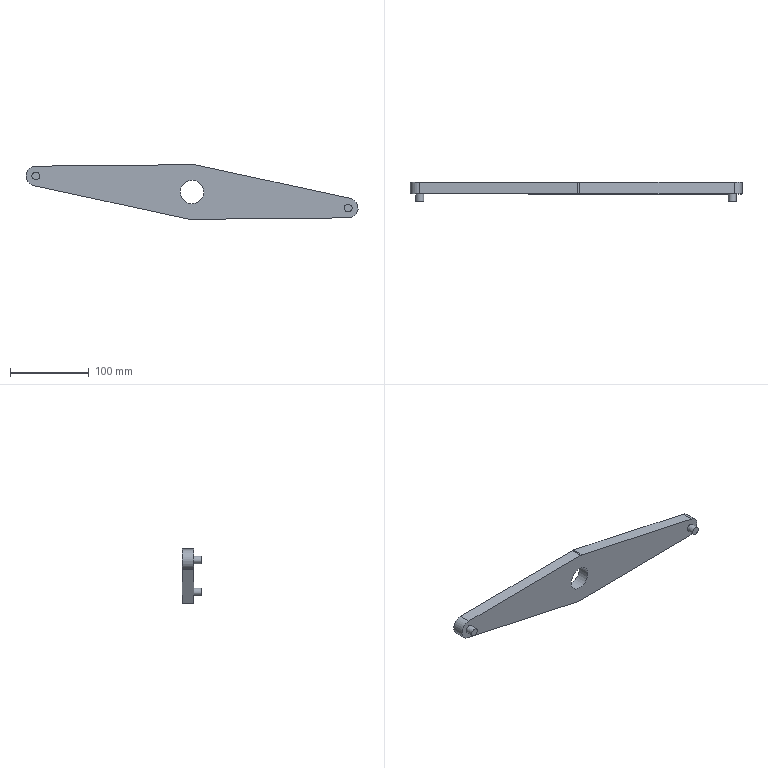Component | NX | 02 | 1 solid | 15 faces | box 422.91 x 25 x 69.61 mm | volume 283802 mm3 | plane 8 | cylinder 7 | commonest cylinder face diameters 25 x2 20 x2 10 x2 30 x1
STEP:
#1=CARTESIAN_POINT('',(0.,0.,0.));
#2=DIRECTION('',(0.,0.,1.));
#3=DIRECTION('',(1.,0.,0.));
#4=AXIS2_PLACEMENT_3D('',#1,#2,#3);
#5=CARTESIAN_POINT('',(-199.074,30.,352.909));
#6=VERTEX_POINT('',#5);
#7=CARTESIAN_POINT('',(-201.609,30.,328.194));
#8=VERTEX_POINT('',#7);
#9=CARTESIAN_POINT('',(-198.956,30.,340.41));
#10=DIRECTION('',(0.,-1.,0.));
#11=DIRECTION('',(-0.9948,0.,0.102));
#12=AXIS2_PLACEMENT_3D('',#9,#10,#11);
#13=CIRCLE('',#12,12.5);
#14=CARTESIAN_POINT('',(-198.956,15.,340.41));
#15=DIRECTION('',(0.,1.,0.));
#16=DIRECTION('',(0.102,0.,0.9948));
#17=AXIS2_PLACEMENT_3D('',#14,#15,#16);
#18=CYLINDRICAL_SURFACE('',#17,12.5);
#19=CARTESIAN_POINT('',(10.996,15.));
#20=DIRECTION('',(-1.,0.));
#21=VECTOR('',#20,1.);
#22=LINE('',#19,#21);
#23=(GEOMETRIC_REPRESENTATION_CONTEXT(2)PARAMETRIC_REPRESENTATION_CONTEXT()REPRESENTATION_CONTEXT('',''));
#24=DEFINITIONAL_REPRESENTATION('',(#22),#23);
#25=PCURVE('',#18,#24);
#26=CARTESIAN_POINT('',(-198.956,30.,340.41));
#27=DIRECTION('',(0.,-1.,0.));
#28=DIRECTION('',(-0.102,0.,-0.9948));
#29=AXIS2_PLACEMENT_3D('',#26,#27,#28);
#30=PLANE('',#29);
#31=CARTESIAN_POINT('',(0.,0.));
#32=DIRECTION('',(-0.,-1.));
#33=AXIS2_PLACEMENT_2D('',#31,#32);
#34=CIRCLE('',#33,12.5);
#35=(GEOMETRIC_REPRESENTATION_CONTEXT(2)PARAMETRIC_REPRESENTATION_CONTEXT()REPRESENTATION_CONTEXT('',''));
#36=DEFINITIONAL_REPRESENTATION('',(#34),#35);
#37=PCURVE('',#30,#36);
#38=SURFACE_CURVE('',#13,(#25,#37),.PCURVE_S1.);
#39=EDGE_CURVE('',#6,#8,#38,.T.);
#40=ORIENTED_EDGE('',*,*,#39,.T.);
#41=CARTESIAN_POINT('',(-201.609,15.,328.194));
#42=VERTEX_POINT('',#41);
#43=CARTESIAN_POINT('',(-201.609,15.,328.194));
#44=DIRECTION('',(0.,1.,0.));
#45=VECTOR('',#44,1.);
#46=LINE('',#43,#45);
#47=CARTESIAN_POINT('',(3.253,0.));
#48=DIRECTION('',(0.,1.));
#49=VECTOR('',#48,1.);
#50=LINE('',#47,#49);
#51=(GEOMETRIC_REPRESENTATION_CONTEXT(2)PARAMETRIC_REPRESENTATION_CONTEXT()REPRESENTATION_CONTEXT('',''));
#52=DEFINITIONAL_REPRESENTATION('',(#50),#51);
#53=PCURVE('',#18,#52);
#54=CARTESIAN_POINT('',(-201.609,15.,328.194));
#55=DIRECTION('',(0.2122,0.,0.9772));
#56=DIRECTION('',(0.9772,0.,-0.2122));
#57=AXIS2_PLACEMENT_3D('',#54,#55,#56);
#58=PLANE('',#57);
#59=CARTESIAN_POINT('',(0.,0.));
#60=DIRECTION('',(0.,1.));
#61=VECTOR('',#60,1.);
#62=LINE('',#59,#61);
#63=(GEOMETRIC_REPRESENTATION_CONTEXT(2)PARAMETRIC_REPRESENTATION_CONTEXT()REPRESENTATION_CONTEXT('',''));
#64=DEFINITIONAL_REPRESENTATION('',(#62),#63);
#65=PCURVE('',#58,#64);
#66=SURFACE_CURVE('',#46,(#53,#65),.PCURVE_S1.);
#67=EDGE_CURVE('',#42,#8,#66,.T.);
#68=ORIENTED_EDGE('',*,*,#67,.F.);
#69=CARTESIAN_POINT('',(-199.074,15.,352.909));
#70=VERTEX_POINT('',#69);
#71=CARTESIAN_POINT('',(-198.956,15.,340.41));
#72=DIRECTION('',(0.,-1.,0.));
#73=DIRECTION('',(-0.9948,0.,0.102));
#74=AXIS2_PLACEMENT_3D('',#71,#72,#73);
#75=CIRCLE('',#74,12.5);
#76=CARTESIAN_POINT('',(10.996,0.));
#77=DIRECTION('',(-1.,0.));
#78=VECTOR('',#77,1.);
#79=LINE('',#76,#78);
#80=(GEOMETRIC_REPRESENTATION_CONTEXT(2)PARAMETRIC_REPRESENTATION_CONTEXT()REPRESENTATION_CONTEXT('',''));
#81=DEFINITIONAL_REPRESENTATION('',(#79),#80);
#82=PCURVE('',#18,#81);
#83=CARTESIAN_POINT('',(-198.956,15.,340.41));
#84=DIRECTION('',(0.,-1.,0.));
#85=DIRECTION('',(-0.102,0.,-0.9948));
#86=AXIS2_PLACEMENT_3D('',#83,#84,#85);
#87=PLANE('',#86);
#88=CARTESIAN_POINT('',(0.,0.));
#89=DIRECTION('',(-0.,-1.));
#90=AXIS2_PLACEMENT_2D('',#88,#89);
#91=CIRCLE('',#90,12.5);
#92=(GEOMETRIC_REPRESENTATION_CONTEXT(2)PARAMETRIC_REPRESENTATION_CONTEXT()REPRESENTATION_CONTEXT('',''));
#93=DEFINITIONAL_REPRESENTATION('',(#91),#92);
#94=PCURVE('',#87,#93);
#95=SURFACE_CURVE('',#75,(#82,#94),.PCURVE_S1.);
#96=EDGE_CURVE('',#70,#42,#95,.T.);
#97=ORIENTED_EDGE('',*,*,#96,.F.);
#98=CARTESIAN_POINT('',(-199.074,15.,352.909));
#99=DIRECTION('',(0.,1.,0.));
#100=VECTOR('',#99,1.);
#101=LINE('',#98,#100);
#102=CARTESIAN_POINT('',(6.172,0.));
#103=DIRECTION('',(0.,1.));
#104=VECTOR('',#103,1.);
#105=LINE('',#102,#104);
#106=(GEOMETRIC_REPRESENTATION_CONTEXT(2)PARAMETRIC_REPRESENTATION_CONTEXT()REPRESENTATION_CONTEXT('',''));
#107=DEFINITIONAL_REPRESENTATION('',(#105),#106);
#108=PCURVE('',#18,#107);
#109=CARTESIAN_POINT('',(3.572,15.,354.817));
#110=DIRECTION('',(0.009416,0.,-1.));
#111=DIRECTION('',(-1.,0.,-0.009416));
#112=AXIS2_PLACEMENT_3D('',#109,#110,#111);
#113=PLANE('',#112);
#114=CARTESIAN_POINT('',(202.654,0.));
#115=DIRECTION('',(0.,1.));
#116=VECTOR('',#115,1.);
#117=LINE('',#114,#116);
#118=(GEOMETRIC_REPRESENTATION_CONTEXT(2)PARAMETRIC_REPRESENTATION_CONTEXT()REPRESENTATION_CONTEXT('',''));
#119=DEFINITIONAL_REPRESENTATION('',(#117),#118);
#120=PCURVE('',#113,#119);
#121=SURFACE_CURVE('',#101,(#108,#120),.PCURVE_S1.);
#122=EDGE_CURVE('',#70,#6,#121,.T.);
#123=ORIENTED_EDGE('',*,*,#122,.T.);
#124=EDGE_LOOP('',(#40,#68,#97,#123));
#125=FACE_BOUND('',#124,.T.);
#126=ADVANCED_FACE('',(#125),#18,.T.);
#127=CARTESIAN_POINT('',(-4.667,30.,285.421));
#128=VERTEX_POINT('',#127);
#129=CARTESIAN_POINT('',(-201.609,30.,328.194));
#130=DIRECTION('',(0.9772,0.,-0.2122));
#131=VECTOR('',#130,1.);
#132=LINE('',#129,#131);
#133=CARTESIAN_POINT('',(0.,15.));
#134=DIRECTION('',(1.,0.));
#135=VECTOR('',#134,1.);
#136=LINE('',#133,#135);
#137=(GEOMETRIC_REPRESENTATION_CONTEXT(2)PARAMETRIC_REPRESENTATION_CONTEXT()REPRESENTATION_CONTEXT('',''));
#138=DEFINITIONAL_REPRESENTATION('',(#136),#137);
#139=PCURVE('',#58,#138);
#140=CARTESIAN_POINT('',(12.422,-1.393));
#141=DIRECTION('',(0.1114,0.9938));
#142=VECTOR('',#141,1.);
#143=LINE('',#140,#142);
#144=(GEOMETRIC_REPRESENTATION_CONTEXT(2)PARAMETRIC_REPRESENTATION_CONTEXT()REPRESENTATION_CONTEXT('',''));
#145=DEFINITIONAL_REPRESENTATION('',(#143),#144);
#146=PCURVE('',#30,#145);
#147=SURFACE_CURVE('',#132,(#139,#146),.PCURVE_S1.);
#148=EDGE_CURVE('',#8,#128,#147,.T.);
#149=ORIENTED_EDGE('',*,*,#148,.T.);
#150=CARTESIAN_POINT('',(-4.667,15.,285.421));
#151=VERTEX_POINT('',#150);
#152=CARTESIAN_POINT('',(-4.667,15.,285.421));
#153=DIRECTION('',(0.,-1.,0.));
#154=VECTOR('',#153,1.);
#155=LINE('',#152,#154);
#156=CARTESIAN_POINT('',(201.533,0.));
#157=DIRECTION('',(0.,-1.));
#158=VECTOR('',#157,1.);
#159=LINE('',#156,#158);
#160=(GEOMETRIC_REPRESENTATION_CONTEXT(2)PARAMETRIC_REPRESENTATION_CONTEXT()REPRESENTATION_CONTEXT('',''));
#161=DEFINITIONAL_REPRESENTATION('',(#159),#160);
#162=PCURVE('',#58,#161);
#163=CARTESIAN_POINT('',(-2.545,15.,295.193));
#164=DIRECTION('',(0.,1.,0.));
#165=DIRECTION('',(0.102,0.,0.9948));
#166=AXIS2_PLACEMENT_3D('',#163,#164,#165);
#167=CYLINDRICAL_SURFACE('',#166,10.);
#168=CARTESIAN_POINT('',(3.253,0.));
#169=DIRECTION('',(0.,-1.));
#170=VECTOR('',#169,1.);
#171=LINE('',#168,#170);
#172=(GEOMETRIC_REPRESENTATION_CONTEXT(2)PARAMETRIC_REPRESENTATION_CONTEXT()REPRESENTATION_CONTEXT('',''));
#173=DEFINITIONAL_REPRESENTATION('',(#171),#172);
#174=PCURVE('',#167,#173);
#175=SURFACE_CURVE('',#155,(#162,#174),.PCURVE_S1.);
#176=EDGE_CURVE('',#128,#151,#175,.T.);
#177=ORIENTED_EDGE('',*,*,#176,.T.);
#178=CARTESIAN_POINT('',(-201.609,15.,328.194));
#179=DIRECTION('',(0.9772,0.,-0.2122));
#180=VECTOR('',#179,1.);
#181=LINE('',#178,#180);
#182=CARTESIAN_POINT('',(0.,0.));
#183=DIRECTION('',(1.,0.));
#184=VECTOR('',#183,1.);
#185=LINE('',#182,#184);
#186=(GEOMETRIC_REPRESENTATION_CONTEXT(2)PARAMETRIC_REPRESENTATION_CONTEXT()REPRESENTATION_CONTEXT('',''));
#187=DEFINITIONAL_REPRESENTATION('',(#185),#186);
#188=PCURVE('',#58,#187);
#189=CARTESIAN_POINT('',(12.422,-1.393));
#190=DIRECTION('',(0.1114,0.9938));
#191=VECTOR('',#190,1.);
#192=LINE('',#189,#191);
#193=(GEOMETRIC_REPRESENTATION_CONTEXT(2)PARAMETRIC_REPRESENTATION_CONTEXT()REPRESENTATION_CONTEXT('',''));
#194=DEFINITIONAL_REPRESENTATION('',(#192),#193);
#195=PCURVE('',#87,#194);
#196=SURFACE_CURVE('',#181,(#188,#195),.PCURVE_S1.);
#197=EDGE_CURVE('',#42,#151,#196,.T.);
#198=ORIENTED_EDGE('',*,*,#197,.F.);
#199=ORIENTED_EDGE('',*,*,#67,.T.);
#200=EDGE_LOOP('',(#149,#177,#198,#199));
#201=FACE_BOUND('',#200,.T.);
#202=ADVANCED_FACE('',(#201),#58,.F.);
#203=CARTESIAN_POINT('',(-2.451,15.,285.193));
#204=VERTEX_POINT('',#203);
#205=CARTESIAN_POINT('',(199.074,15.,287.091));
#206=VERTEX_POINT('',#205);
#207=CARTESIAN_POINT('',(-3.572,15.,285.183));
#208=DIRECTION('',(1.,0.,0.009416));
#209=VECTOR('',#208,1.);
#210=LINE('',#207,#209);
#211=CARTESIAN_POINT('',(-3.572,15.,285.183));
#212=DIRECTION('',(-0.009416,0.,1.));
#213=DIRECTION('',(1.,0.,0.009416));
#214=AXIS2_PLACEMENT_3D('',#211,#212,#213);
#215=PLANE('',#214);
#216=CARTESIAN_POINT('',(0.,0.));
#217=DIRECTION('',(1.,0.));
#218=VECTOR('',#217,1.);
#219=LINE('',#216,#218);
#220=(GEOMETRIC_REPRESENTATION_CONTEXT(2)PARAMETRIC_REPRESENTATION_CONTEXT()REPRESENTATION_CONTEXT('',''));
#221=DEFINITIONAL_REPRESENTATION('',(#219),#220);
#222=PCURVE('',#215,#221);
#223=CARTESIAN_POINT('',(35.,200.));
#224=DIRECTION('',(-0.1114,0.9938));
#225=VECTOR('',#224,1.);
#226=LINE('',#223,#225);
#227=(GEOMETRIC_REPRESENTATION_CONTEXT(2)PARAMETRIC_REPRESENTATION_CONTEXT()REPRESENTATION_CONTEXT('',''));
#228=DEFINITIONAL_REPRESENTATION('',(#226),#227);
#229=PCURVE('',#87,#228);
#230=SURFACE_CURVE('',#210,(#222,#229),.PCURVE_S1.);
#231=EDGE_CURVE('',#204,#206,#230,.T.);
#232=ORIENTED_EDGE('',*,*,#231,.F.);
#233=CARTESIAN_POINT('',(-2.451,30.,285.193));
#234=VERTEX_POINT('',#233);
#235=CARTESIAN_POINT('',(-2.451,15.,285.193));
#236=DIRECTION('',(0.,1.,0.));
#237=VECTOR('',#236,1.);
#238=LINE('',#235,#237);
#239=CARTESIAN_POINT('',(1.121,0.));
#240=DIRECTION('',(0.,1.));
#241=VECTOR('',#240,1.);
#242=LINE('',#239,#241);
#243=(GEOMETRIC_REPRESENTATION_CONTEXT(2)PARAMETRIC_REPRESENTATION_CONTEXT()REPRESENTATION_CONTEXT('',''));
#244=DEFINITIONAL_REPRESENTATION('',(#242),#243);
#245=PCURVE('',#215,#244);
#246=CARTESIAN_POINT('',(3.03,0.));
#247=DIRECTION('',(0.,1.));
#248=VECTOR('',#247,1.);
#249=LINE('',#246,#248);
#250=(GEOMETRIC_REPRESENTATION_CONTEXT(2)PARAMETRIC_REPRESENTATION_CONTEXT()REPRESENTATION_CONTEXT('',''));
#251=DEFINITIONAL_REPRESENTATION('',(#249),#250);
#252=PCURVE('',#167,#251);
#253=SURFACE_CURVE('',#238,(#245,#252),.PCURVE_S1.);
#254=EDGE_CURVE('',#204,#234,#253,.T.);
#255=ORIENTED_EDGE('',*,*,#254,.T.);
#256=CARTESIAN_POINT('',(199.074,30.,287.091));
#257=VERTEX_POINT('',#256);
#258=CARTESIAN_POINT('',(-3.572,30.,285.183));
#259=DIRECTION('',(1.,0.,0.009416));
#260=VECTOR('',#259,1.);
#261=LINE('',#258,#260);
#262=CARTESIAN_POINT('',(0.,15.));
#263=DIRECTION('',(1.,0.));
#264=VECTOR('',#263,1.);
#265=LINE('',#262,#264);
#266=(GEOMETRIC_REPRESENTATION_CONTEXT(2)PARAMETRIC_REPRESENTATION_CONTEXT()REPRESENTATION_CONTEXT('',''));
#267=DEFINITIONAL_REPRESENTATION('',(#265),#266);
#268=PCURVE('',#215,#267);
#269=CARTESIAN_POINT('',(35.,200.));
#270=DIRECTION('',(-0.1114,0.9938));
#271=VECTOR('',#270,1.);
#272=LINE('',#269,#271);
#273=(GEOMETRIC_REPRESENTATION_CONTEXT(2)PARAMETRIC_REPRESENTATION_CONTEXT()REPRESENTATION_CONTEXT('',''));
#274=DEFINITIONAL_REPRESENTATION('',(#272),#273);
#275=PCURVE('',#30,#274);
#276=SURFACE_CURVE('',#261,(#268,#275),.PCURVE_S1.);
#277=EDGE_CURVE('',#234,#257,#276,.T.);
#278=ORIENTED_EDGE('',*,*,#277,.T.);
#279=CARTESIAN_POINT('',(199.074,15.,287.091));
#280=DIRECTION('',(0.,1.,0.));
#281=VECTOR('',#280,1.);
#282=LINE('',#279,#281);
#283=CARTESIAN_POINT('',(202.654,0.));
#284=DIRECTION('',(0.,1.));
#285=VECTOR('',#284,1.);
#286=LINE('',#283,#285);
#287=(GEOMETRIC_REPRESENTATION_CONTEXT(2)PARAMETRIC_REPRESENTATION_CONTEXT()REPRESENTATION_CONTEXT('',''));
#288=DEFINITIONAL_REPRESENTATION('',(#286),#287);
#289=PCURVE('',#215,#288);
#290=CARTESIAN_POINT('',(198.956,15.,299.59));
#291=DIRECTION('',(0.,1.,0.));
#292=DIRECTION('',(0.102,0.,0.9948));
#293=AXIS2_PLACEMENT_3D('',#290,#291,#292);
#294=CYLINDRICAL_SURFACE('',#293,12.5);
#295=CARTESIAN_POINT('',(3.03,0.));
#296=DIRECTION('',(0.,1.));
#297=VECTOR('',#296,1.);
#298=LINE('',#295,#297);
#299=(GEOMETRIC_REPRESENTATION_CONTEXT(2)PARAMETRIC_REPRESENTATION_CONTEXT()REPRESENTATION_CONTEXT('',''));
#300=DEFINITIONAL_REPRESENTATION('',(#298),#299);
#301=PCURVE('',#294,#300);
#302=SURFACE_CURVE('',#282,(#289,#301),.PCURVE_S1.);
#303=EDGE_CURVE('',#206,#257,#302,.T.);
#304=ORIENTED_EDGE('',*,*,#303,.F.);
#305=EDGE_LOOP('',(#232,#255,#278,#304));
#306=FACE_BOUND('',#305,.T.);
#307=ADVANCED_FACE('',(#306),#215,.F.);
#308=CARTESIAN_POINT('',(201.609,30.,311.806));
#309=VERTEX_POINT('',#308);
#310=CARTESIAN_POINT('',(198.956,30.,299.59));
#311=DIRECTION('',(0.,-1.,0.));
#312=DIRECTION('',(0.9948,0.,-0.102));
#313=AXIS2_PLACEMENT_3D('',#310,#311,#312);
#314=CIRCLE('',#313,12.5);
#315=CARTESIAN_POINT('',(7.854,15.));
#316=DIRECTION('',(-1.,0.));
#317=VECTOR('',#316,1.);
#318=LINE('',#315,#317);
#319=(GEOMETRIC_REPRESENTATION_CONTEXT(2)PARAMETRIC_REPRESENTATION_CONTEXT()REPRESENTATION_CONTEXT('',''));
#320=DEFINITIONAL_REPRESENTATION('',(#318),#319);
#321=PCURVE('',#294,#320);
#322=CARTESIAN_POINT('',(-0.,400.));
#323=DIRECTION('',(0.,1.));
#324=AXIS2_PLACEMENT_2D('',#322,#323);
#325=CIRCLE('',#324,12.5);
#326=(GEOMETRIC_REPRESENTATION_CONTEXT(2)PARAMETRIC_REPRESENTATION_CONTEXT()REPRESENTATION_CONTEXT('',''));
#327=DEFINITIONAL_REPRESENTATION('',(#325),#326);
#328=PCURVE('',#30,#327);
#329=SURFACE_CURVE('',#314,(#321,#328),.PCURVE_S1.);
#330=EDGE_CURVE('',#257,#309,#329,.T.);
#331=ORIENTED_EDGE('',*,*,#330,.T.);
#332=CARTESIAN_POINT('',(201.609,15.,311.806));
#333=VERTEX_POINT('',#332);
#334=CARTESIAN_POINT('',(201.609,15.,311.806));
#335=DIRECTION('',(0.,1.,0.));
#336=VECTOR('',#335,1.);
#337=LINE('',#334,#336);
#338=CARTESIAN_POINT('',(0.1116,0.));
#339=DIRECTION('',(0.,1.));
#340=VECTOR('',#339,1.);
#341=LINE('',#338,#340);
#342=(GEOMETRIC_REPRESENTATION_CONTEXT(2)PARAMETRIC_REPRESENTATION_CONTEXT()REPRESENTATION_CONTEXT('',''));
#343=DEFINITIONAL_REPRESENTATION('',(#341),#342);
#344=PCURVE('',#294,#343);
#345=CARTESIAN_POINT('',(201.609,15.,311.806));
#346=DIRECTION('',(-0.2122,0.,-0.9772));
#347=DIRECTION('',(-0.9772,0.,0.2122));
#348=AXIS2_PLACEMENT_3D('',#345,#346,#347);
#349=PLANE('',#348);
#350=CARTESIAN_POINT('',(0.,0.));
#351=DIRECTION('',(0.,1.));
#352=VECTOR('',#351,1.);
#353=LINE('',#350,#352);
#354=(GEOMETRIC_REPRESENTATION_CONTEXT(2)PARAMETRIC_REPRESENTATION_CONTEXT()REPRESENTATION_CONTEXT('',''));
#355=DEFINITIONAL_REPRESENTATION('',(#353),#354);
#356=PCURVE('',#349,#355);
#357=SURFACE_CURVE('',#337,(#344,#356),.PCURVE_S1.);
#358=EDGE_CURVE('',#333,#309,#357,.T.);
#359=ORIENTED_EDGE('',*,*,#358,.F.);
#360=CARTESIAN_POINT('',(198.956,15.,299.59));
#361=DIRECTION('',(0.,-1.,0.));
#362=DIRECTION('',(0.9948,0.,-0.102));
#363=AXIS2_PLACEMENT_3D('',#360,#361,#362);
#364=CIRCLE('',#363,12.5);
#365=CARTESIAN_POINT('',(7.854,0.));
#366=DIRECTION('',(-1.,0.));
#367=VECTOR('',#366,1.);
#368=LINE('',#365,#367);
#369=(GEOMETRIC_REPRESENTATION_CONTEXT(2)PARAMETRIC_REPRESENTATION_CONTEXT()REPRESENTATION_CONTEXT('',''));
#370=DEFINITIONAL_REPRESENTATION('',(#368),#369);
#371=PCURVE('',#294,#370);
#372=CARTESIAN_POINT('',(-0.,400.));
#373=DIRECTION('',(0.,1.));
#374=AXIS2_PLACEMENT_2D('',#372,#373);
#375=CIRCLE('',#374,12.5);
#376=(GEOMETRIC_REPRESENTATION_CONTEXT(2)PARAMETRIC_REPRESENTATION_CONTEXT()REPRESENTATION_CONTEXT('',''));
#377=DEFINITIONAL_REPRESENTATION('',(#375),#376);
#378=PCURVE('',#87,#377);
#379=SURFACE_CURVE('',#364,(#371,#378),.PCURVE_S1.);
#380=EDGE_CURVE('',#206,#333,#379,.T.);
#381=ORIENTED_EDGE('',*,*,#380,.F.);
#382=ORIENTED_EDGE('',*,*,#303,.T.);
#383=EDGE_LOOP('',(#331,#359,#381,#382));
#384=FACE_BOUND('',#383,.T.);
#385=ADVANCED_FACE('',(#384),#294,.T.);
#386=CARTESIAN_POINT('',(4.667,30.,354.579));
#387=VERTEX_POINT('',#386);
#388=CARTESIAN_POINT('',(201.609,30.,311.806));
#389=DIRECTION('',(-0.9772,0.,0.2122));
#390=VECTOR('',#389,1.);
#391=LINE('',#388,#390);
#392=CARTESIAN_POINT('',(0.,15.));
#393=DIRECTION('',(1.,0.));
#394=VECTOR('',#393,1.);
#395=LINE('',#392,#394);
#396=(GEOMETRIC_REPRESENTATION_CONTEXT(2)PARAMETRIC_REPRESENTATION_CONTEXT()REPRESENTATION_CONTEXT('',''));
#397=DEFINITIONAL_REPRESENTATION('',(#395),#396);
#398=PCURVE('',#349,#397);
#399=CARTESIAN_POINT('',(-12.422,401.393));
#400=DIRECTION('',(-0.1114,-0.9938));
#401=VECTOR('',#400,1.);
#402=LINE('',#399,#401);
#403=(GEOMETRIC_REPRESENTATION_CONTEXT(2)PARAMETRIC_REPRESENTATION_CONTEXT()REPRESENTATION_CONTEXT('',''));
#404=DEFINITIONAL_REPRESENTATION('',(#402),#403);
#405=PCURVE('',#30,#404);
#406=SURFACE_CURVE('',#391,(#398,#405),.PCURVE_S1.);
#407=EDGE_CURVE('',#309,#387,#406,.T.);
#408=ORIENTED_EDGE('',*,*,#407,.T.);
#409=CARTESIAN_POINT('',(4.667,15.,354.579));
#410=VERTEX_POINT('',#409);
#411=CARTESIAN_POINT('',(4.667,15.,354.579));
#412=DIRECTION('',(0.,-1.,0.));
#413=VECTOR('',#412,1.);
#414=LINE('',#411,#413);
#415=CARTESIAN_POINT('',(201.533,0.));
#416=DIRECTION('',(0.,-1.));
#417=VECTOR('',#416,1.);
#418=LINE('',#415,#417);
#419=(GEOMETRIC_REPRESENTATION_CONTEXT(2)PARAMETRIC_REPRESENTATION_CONTEXT()REPRESENTATION_CONTEXT('',''));
#420=DEFINITIONAL_REPRESENTATION('',(#418),#419);
#421=PCURVE('',#349,#420);
#422=CARTESIAN_POINT('',(2.545,15.,344.807));
#423=DIRECTION('',(0.,1.,0.));
#424=DIRECTION('',(0.102,0.,0.9948));
#425=AXIS2_PLACEMENT_3D('',#422,#423,#424);
#426=CYLINDRICAL_SURFACE('',#425,10.);
#427=CARTESIAN_POINT('',(0.1116,0.));
#428=DIRECTION('',(0.,-1.));
#429=VECTOR('',#428,1.);
#430=LINE('',#427,#429);
#431=(GEOMETRIC_REPRESENTATION_CONTEXT(2)PARAMETRIC_REPRESENTATION_CONTEXT()REPRESENTATION_CONTEXT('',''));
#432=DEFINITIONAL_REPRESENTATION('',(#430),#431);
#433=PCURVE('',#426,#432);
#434=SURFACE_CURVE('',#414,(#421,#433),.PCURVE_S1.);
#435=EDGE_CURVE('',#387,#410,#434,.T.);
#436=ORIENTED_EDGE('',*,*,#435,.T.);
#437=CARTESIAN_POINT('',(201.609,15.,311.806));
#438=DIRECTION('',(-0.9772,0.,0.2122));
#439=VECTOR('',#438,1.);
#440=LINE('',#437,#439);
#441=CARTESIAN_POINT('',(0.,0.));
#442=DIRECTION('',(1.,0.));
#443=VECTOR('',#442,1.);
#444=LINE('',#441,#443);
#445=(GEOMETRIC_REPRESENTATION_CONTEXT(2)PARAMETRIC_REPRESENTATION_CONTEXT()REPRESENTATION_CONTEXT('',''));
#446=DEFINITIONAL_REPRESENTATION('',(#444),#445);
#447=PCURVE('',#349,#446);
#448=CARTESIAN_POINT('',(-12.422,401.393));
#449=DIRECTION('',(-0.1114,-0.9938));
#450=VECTOR('',#449,1.);
#451=LINE('',#448,#450);
#452=(GEOMETRIC_REPRESENTATION_CONTEXT(2)PARAMETRIC_REPRESENTATION_CONTEXT()REPRESENTATION_CONTEXT('',''));
#453=DEFINITIONAL_REPRESENTATION('',(#451),#452);
#454=PCURVE('',#87,#453);
#455=SURFACE_CURVE('',#440,(#447,#454),.PCURVE_S1.);
#456=EDGE_CURVE('',#333,#410,#455,.T.);
#457=ORIENTED_EDGE('',*,*,#456,.F.);
#458=ORIENTED_EDGE('',*,*,#358,.T.);
#459=EDGE_LOOP('',(#408,#436,#457,#458));
#460=FACE_BOUND('',#459,.T.);
#461=ADVANCED_FACE('',(#460),#349,.F.);
#462=CARTESIAN_POINT('',(2.451,15.,354.807));
#463=VERTEX_POINT('',#462);
#464=CARTESIAN_POINT('',(3.572,15.,354.817));
#465=DIRECTION('',(-1.,0.,-0.009416));
#466=VECTOR('',#465,1.);
#467=LINE('',#464,#466);
#468=CARTESIAN_POINT('',(0.,0.));
#469=DIRECTION('',(1.,0.));
#470=VECTOR('',#469,1.);
#471=LINE('',#468,#470);
#472=(GEOMETRIC_REPRESENTATION_CONTEXT(2)PARAMETRIC_REPRESENTATION_CONTEXT()REPRESENTATION_CONTEXT('',''));
#473=DEFINITIONAL_REPRESENTATION('',(#471),#472);
#474=PCURVE('',#113,#473);
#475=CARTESIAN_POINT('',(-35.,200.));
#476=DIRECTION('',(0.1114,-0.9938));
#477=VECTOR('',#476,1.);
#478=LINE('',#475,#477);
#479=(GEOMETRIC_REPRESENTATION_CONTEXT(2)PARAMETRIC_REPRESENTATION_CONTEXT()REPRESENTATION_CONTEXT('',''));
#480=DEFINITIONAL_REPRESENTATION('',(#478),#479);
#481=PCURVE('',#87,#480);
#482=SURFACE_CURVE('',#467,(#474,#481),.PCURVE_S1.);
#483=EDGE_CURVE('',#463,#70,#482,.T.);
#484=ORIENTED_EDGE('',*,*,#483,.F.);
#485=CARTESIAN_POINT('',(2.451,30.,354.807));
#486=VERTEX_POINT('',#485);
#487=CARTESIAN_POINT('',(2.451,15.,354.807));
#488=DIRECTION('',(0.,1.,0.));
#489=VECTOR('',#488,1.);
#490=LINE('',#487,#489);
#491=CARTESIAN_POINT('',(1.121,0.));
#492=DIRECTION('',(0.,1.));
#493=VECTOR('',#492,1.);
#494=LINE('',#491,#493);
#495=(GEOMETRIC_REPRESENTATION_CONTEXT(2)PARAMETRIC_REPRESENTATION_CONTEXT()REPRESENTATION_CONTEXT('',''));
#496=DEFINITIONAL_REPRESENTATION('',(#494),#495);
#497=PCURVE('',#113,#496);
#498=CARTESIAN_POINT('',(-0.1116,0.));
#499=DIRECTION('',(0.,1.));
#500=VECTOR('',#499,1.);
#501=LINE('',#498,#500);
#502=(GEOMETRIC_REPRESENTATION_CONTEXT(2)PARAMETRIC_REPRESENTATION_CONTEXT()REPRESENTATION_CONTEXT('',''));
#503=DEFINITIONAL_REPRESENTATION('',(#501),#502);
#504=PCURVE('',#426,#503);
#505=SURFACE_CURVE('',#490,(#497,#504),.PCURVE_S1.);
#506=EDGE_CURVE('',#463,#486,#505,.T.);
#507=ORIENTED_EDGE('',*,*,#506,.T.);
#508=CARTESIAN_POINT('',(3.572,30.,354.817));
#509=DIRECTION('',(-1.,0.,-0.009416));
#510=VECTOR('',#509,1.);
#511=LINE('',#508,#510);
#512=CARTESIAN_POINT('',(0.,15.));
#513=DIRECTION('',(1.,0.));
#514=VECTOR('',#513,1.);
#515=LINE('',#512,#514);
#516=(GEOMETRIC_REPRESENTATION_CONTEXT(2)PARAMETRIC_REPRESENTATION_CONTEXT()REPRESENTATION_CONTEXT('',''));
#517=DEFINITIONAL_REPRESENTATION('',(#515),#516);
#518=PCURVE('',#113,#517);
#519=CARTESIAN_POINT('',(-35.,200.));
#520=DIRECTION('',(0.1114,-0.9938));
#521=VECTOR('',#520,1.);
#522=LINE('',#519,#521);
#523=(GEOMETRIC_REPRESENTATION_CONTEXT(2)PARAMETRIC_REPRESENTATION_CONTEXT()REPRESENTATION_CONTEXT('',''));
#524=DEFINITIONAL_REPRESENTATION('',(#522),#523);
#525=PCURVE('',#30,#524);
#526=SURFACE_CURVE('',#511,(#518,#525),.PCURVE_S1.);
#527=EDGE_CURVE('',#486,#6,#526,.T.);
#528=ORIENTED_EDGE('',*,*,#527,.T.);
#529=ORIENTED_EDGE('',*,*,#122,.F.);
#530=EDGE_LOOP('',(#484,#507,#528,#529));
#531=FACE_BOUND('',#530,.T.);
#532=ADVANCED_FACE('',(#531),#113,.F.);
#533=CARTESIAN_POINT('',(203.93,15.,299.08));
#534=VERTEX_POINT('',#533);
#535=CARTESIAN_POINT('',(198.956,15.,299.59));
#536=DIRECTION('',(0.,-1.,0.));
#537=DIRECTION('',(0.9948,0.,-0.102));
#538=AXIS2_PLACEMENT_3D('',#535,#536,#537);
#539=CIRCLE('',#538,5.);
#540=CARTESIAN_POINT('',(-0.,400.));
#541=DIRECTION('',(-0.,1.));
#542=AXIS2_PLACEMENT_2D('',#540,#541);
#543=CIRCLE('',#542,5.);
#544=(GEOMETRIC_REPRESENTATION_CONTEXT(2)PARAMETRIC_REPRESENTATION_CONTEXT()REPRESENTATION_CONTEXT('',''));
#545=DEFINITIONAL_REPRESENTATION('',(#543),#544);
#546=PCURVE('',#87,#545);
#547=CARTESIAN_POINT('',(198.956,5.,299.59));
#548=DIRECTION('',(0.,1.,0.));
#549=DIRECTION('',(0.102,0.,0.9948));
#550=AXIS2_PLACEMENT_3D('',#547,#548,#549);
#551=CYLINDRICAL_SURFACE('',#550,5.);
#552=CARTESIAN_POINT('',(7.854,10.));
#553=DIRECTION('',(-1.,0.));
#554=VECTOR('',#553,1.);
#555=LINE('',#552,#554);
#556=(GEOMETRIC_REPRESENTATION_CONTEXT(2)PARAMETRIC_REPRESENTATION_CONTEXT()REPRESENTATION_CONTEXT('',''));
#557=DEFINITIONAL_REPRESENTATION('',(#555),#556);
#558=PCURVE('',#551,#557);
#559=SURFACE_CURVE('',#539,(#546,#558),.PCURVE_S1.);
#560=EDGE_CURVE('',#534,#534,#559,.T.);
#561=ORIENTED_EDGE('',*,*,#560,.F.);
#562=EDGE_LOOP('',(#561));
#563=FACE_BOUND('',#562,.T.);
#564=CARTESIAN_POINT('',(-193.982,15.,339.899));
#565=VERTEX_POINT('',#564);
#566=CARTESIAN_POINT('',(-198.956,15.,340.41));
#567=DIRECTION('',(0.,-1.,0.));
#568=DIRECTION('',(0.9948,0.,-0.102));
#569=AXIS2_PLACEMENT_3D('',#566,#567,#568);
#570=CIRCLE('',#569,5.);
#571=CARTESIAN_POINT('',(0.,0.));
#572=DIRECTION('',(-0.,1.));
#573=AXIS2_PLACEMENT_2D('',#571,#572);
#574=CIRCLE('',#573,5.);
#575=(GEOMETRIC_REPRESENTATION_CONTEXT(2)PARAMETRIC_REPRESENTATION_CONTEXT()REPRESENTATION_CONTEXT('',''));
#576=DEFINITIONAL_REPRESENTATION('',(#574),#575);
#577=PCURVE('',#87,#576);
#578=CARTESIAN_POINT('',(-198.956,5.,340.41));
#579=DIRECTION('',(0.,1.,0.));
#580=DIRECTION('',(0.102,0.,0.9948));
#581=AXIS2_PLACEMENT_3D('',#578,#579,#580);
#582=CYLINDRICAL_SURFACE('',#581,5.);
#583=CARTESIAN_POINT('',(7.854,10.));
#584=DIRECTION('',(-1.,0.));
#585=VECTOR('',#584,1.);
#586=LINE('',#583,#585);
#587=(GEOMETRIC_REPRESENTATION_CONTEXT(2)PARAMETRIC_REPRESENTATION_CONTEXT()REPRESENTATION_CONTEXT('',''));
#588=DEFINITIONAL_REPRESENTATION('',(#586),#587);
#589=PCURVE('',#582,#588);
#590=SURFACE_CURVE('',#570,(#577,#589),.PCURVE_S1.);
#591=EDGE_CURVE('',#565,#565,#590,.T.);
#592=ORIENTED_EDGE('',*,*,#591,.F.);
#593=EDGE_LOOP('',(#592));
#594=FACE_BOUND('',#593,.T.);
#595=CARTESIAN_POINT('',(14.922,15.,318.469));
#596=VERTEX_POINT('',#595);
#597=CARTESIAN_POINT('',(0.,15.,320.));
#598=DIRECTION('',(0.,1.,0.));
#599=DIRECTION('',(0.9948,0.,-0.102));
#600=AXIS2_PLACEMENT_3D('',#597,#598,#599);
#601=CIRCLE('',#600,15.);
#602=CARTESIAN_POINT('',(-0.,215.));
#603=CARTESIAN_POINT('',(25.981,215.));
#604=CARTESIAN_POINT('',(12.99,192.5));
#605=CARTESIAN_POINT('',(-0.,170.));
#606=CARTESIAN_POINT('',(-12.99,192.5));
#607=CARTESIAN_POINT('',(-25.981,215.));
#608=CARTESIAN_POINT('',(-0.,215.));
#609=(BOUNDED_CURVE()B_SPLINE_CURVE(2,(#602,#603,#604,#605,#606,#607,#608),.UNSPECIFIED.,.T.,.F.)B_SPLINE_CURVE_WITH_KNOTS((1,2,2,2,2,1),(-2.094,0.,2.094,4.189,6.283,8.378),.UNSPECIFIED.)CURVE()GEOMETRIC_REPRESENTATION_ITEM()RATIONAL_B_SPLINE_CURVE((1.,0.5,1.,0.5,1.,0.5,1.))REPRESENTATION_ITEM(''));
#610=(GEOMETRIC_REPRESENTATION_CONTEXT(2)PARAMETRIC_REPRESENTATION_CONTEXT()REPRESENTATION_CONTEXT('',''));
#611=DEFINITIONAL_REPRESENTATION('',(#609),#610);
#612=PCURVE('',#87,#611);
#613=CARTESIAN_POINT('',(0.,15.,320.));
#614=DIRECTION('',(0.,1.,0.));
#615=DIRECTION('',(0.102,0.,0.9948));
#616=AXIS2_PLACEMENT_3D('',#613,#614,#615);
#617=CYLINDRICAL_SURFACE('',#616,15.);
#618=CARTESIAN_POINT('',(1.571,0.));
#619=DIRECTION('',(1.,0.));
#620=VECTOR('',#619,1.);
#621=LINE('',#618,#620);
#622=(GEOMETRIC_REPRESENTATION_CONTEXT(2)PARAMETRIC_REPRESENTATION_CONTEXT()REPRESENTATION_CONTEXT('',''));
#623=DEFINITIONAL_REPRESENTATION('',(#621),#622);
#624=PCURVE('',#617,#623);
#625=SURFACE_CURVE('',#601,(#612,#624),.PCURVE_S1.);
#626=EDGE_CURVE('',#596,#596,#625,.T.);
#627=ORIENTED_EDGE('',*,*,#626,.T.);
#628=EDGE_LOOP('',(#627));
#629=FACE_BOUND('',#628,.T.);
#630=ORIENTED_EDGE('',*,*,#456,.T.);
#631=CARTESIAN_POINT('',(2.545,15.,344.807));
#632=DIRECTION('',(0.,-1.,0.));
#633=DIRECTION('',(-0.102,0.,-0.9948));
#634=AXIS2_PLACEMENT_3D('',#631,#632,#633);
#635=CIRCLE('',#634,10.);
#636=CARTESIAN_POINT('',(-24.937,200.));
#637=DIRECTION('',(1.,-0.));
#638=AXIS2_PLACEMENT_2D('',#636,#637);
#639=CIRCLE('',#638,10.);
#640=(GEOMETRIC_REPRESENTATION_CONTEXT(2)PARAMETRIC_REPRESENTATION_CONTEXT()REPRESENTATION_CONTEXT('',''));
#641=DEFINITIONAL_REPRESENTATION('',(#639),#640);
#642=PCURVE('',#87,#641);
#643=CARTESIAN_POINT('',(3.142,0.));
#644=DIRECTION('',(-1.,0.));
#645=VECTOR('',#644,1.);
#646=LINE('',#643,#645);
#647=(GEOMETRIC_REPRESENTATION_CONTEXT(2)PARAMETRIC_REPRESENTATION_CONTEXT()REPRESENTATION_CONTEXT('',''));
#648=DEFINITIONAL_REPRESENTATION('',(#646),#647);
#649=PCURVE('',#426,#648);
#650=SURFACE_CURVE('',#635,(#642,#649),.PCURVE_S1.);
#651=EDGE_CURVE('',#410,#463,#650,.T.);
#652=ORIENTED_EDGE('',*,*,#651,.T.);
#653=ORIENTED_EDGE('',*,*,#483,.T.);
#654=ORIENTED_EDGE('',*,*,#96,.T.);
#655=ORIENTED_EDGE('',*,*,#197,.T.);
#656=CARTESIAN_POINT('',(-2.545,15.,295.193));
#657=DIRECTION('',(0.,-1.,0.));
#658=DIRECTION('',(-0.102,0.,-0.9948));
#659=AXIS2_PLACEMENT_3D('',#656,#657,#658);
#660=CIRCLE('',#659,10.);
#661=CARTESIAN_POINT('',(24.937,200.));
#662=DIRECTION('',(1.,-0.));
#663=AXIS2_PLACEMENT_2D('',#661,#662);
#664=CIRCLE('',#663,10.);
#665=(GEOMETRIC_REPRESENTATION_CONTEXT(2)PARAMETRIC_REPRESENTATION_CONTEXT()REPRESENTATION_CONTEXT('',''));
#666=DEFINITIONAL_REPRESENTATION('',(#664),#665);
#667=PCURVE('',#87,#666);
#668=CARTESIAN_POINT('',(9.425,0.));
#669=DIRECTION('',(-1.,0.));
#670=VECTOR('',#669,1.);
#671=LINE('',#668,#670);
#672=(GEOMETRIC_REPRESENTATION_CONTEXT(2)PARAMETRIC_REPRESENTATION_CONTEXT()REPRESENTATION_CONTEXT('',''));
#673=DEFINITIONAL_REPRESENTATION('',(#671),#672);
#674=PCURVE('',#167,#673);
#675=SURFACE_CURVE('',#660,(#667,#674),.PCURVE_S1.);
#676=EDGE_CURVE('',#151,#204,#675,.T.);
#677=ORIENTED_EDGE('',*,*,#676,.T.);
#678=ORIENTED_EDGE('',*,*,#231,.T.);
#679=ORIENTED_EDGE('',*,*,#380,.T.);
#680=EDGE_LOOP('',(#630,#652,#653,#654,#655,#677,#678,#679));
#681=FACE_BOUND('',#680,.T.);
#682=ADVANCED_FACE('',(#563,#594,#629,#681),#87,.T.);
#683=CARTESIAN_POINT('',(14.922,30.,318.469));
#684=VERTEX_POINT('',#683);
#685=CARTESIAN_POINT('',(0.,30.,320.));
#686=DIRECTION('',(0.,1.,0.));
#687=DIRECTION('',(0.9948,0.,-0.102));
#688=AXIS2_PLACEMENT_3D('',#685,#686,#687);
#689=CIRCLE('',#688,15.);
#690=CARTESIAN_POINT('',(-0.,215.));
#691=CARTESIAN_POINT('',(25.981,215.));
#692=CARTESIAN_POINT('',(12.99,192.5));
#693=CARTESIAN_POINT('',(-0.,170.));
#694=CARTESIAN_POINT('',(-12.99,192.5));
#695=CARTESIAN_POINT('',(-25.981,215.));
#696=CARTESIAN_POINT('',(-0.,215.));
#697=(BOUNDED_CURVE()B_SPLINE_CURVE(2,(#690,#691,#692,#693,#694,#695,#696),.UNSPECIFIED.,.T.,.F.)B_SPLINE_CURVE_WITH_KNOTS((1,2,2,2,2,1),(-2.094,0.,2.094,4.189,6.283,8.378),.UNSPECIFIED.)CURVE()GEOMETRIC_REPRESENTATION_ITEM()RATIONAL_B_SPLINE_CURVE((1.,0.5,1.,0.5,1.,0.5,1.))REPRESENTATION_ITEM(''));
#698=(GEOMETRIC_REPRESENTATION_CONTEXT(2)PARAMETRIC_REPRESENTATION_CONTEXT()REPRESENTATION_CONTEXT('',''));
#699=DEFINITIONAL_REPRESENTATION('',(#697),#698);
#700=PCURVE('',#30,#699);
#701=CARTESIAN_POINT('',(1.571,15.));
#702=DIRECTION('',(1.,0.));
#703=VECTOR('',#702,1.);
#704=LINE('',#701,#703);
#705=(GEOMETRIC_REPRESENTATION_CONTEXT(2)PARAMETRIC_REPRESENTATION_CONTEXT()REPRESENTATION_CONTEXT('',''));
#706=DEFINITIONAL_REPRESENTATION('',(#704),#705);
#707=PCURVE('',#617,#706);
#708=SURFACE_CURVE('',#689,(#700,#707),.PCURVE_S1.);
#709=EDGE_CURVE('',#684,#684,#708,.T.);
#710=ORIENTED_EDGE('',*,*,#709,.F.);
#711=EDGE_LOOP('',(#710));
#712=FACE_BOUND('',#711,.T.);
#713=ORIENTED_EDGE('',*,*,#527,.F.);
#714=CARTESIAN_POINT('',(2.545,30.,344.807));
#715=DIRECTION('',(0.,1.,0.));
#716=DIRECTION('',(-0.102,0.,-0.9948));
#717=AXIS2_PLACEMENT_3D('',#714,#715,#716);
#718=CIRCLE('',#717,10.);
#719=CARTESIAN_POINT('',(-14.937,200.));
#720=CARTESIAN_POINT('',(-14.937,182.679));
#721=CARTESIAN_POINT('',(-29.937,191.34));
#722=CARTESIAN_POINT('',(-44.937,200.));
#723=CARTESIAN_POINT('',(-29.937,208.66));
#724=CARTESIAN_POINT('',(-14.937,217.321));
#725=CARTESIAN_POINT('',(-14.937,200.));
#726=(BOUNDED_CURVE()B_SPLINE_CURVE(2,(#719,#720,#721,#722,#723,#724,#725),.UNSPECIFIED.,.T.,.F.)B_SPLINE_CURVE_WITH_KNOTS((1,2,2,2,2,1),(-2.094,0.,2.094,4.189,6.283,8.378),.UNSPECIFIED.)CURVE()GEOMETRIC_REPRESENTATION_ITEM()RATIONAL_B_SPLINE_CURVE((1.,0.5,1.,0.5,1.,0.5,1.))REPRESENTATION_ITEM(''));
#727=(GEOMETRIC_REPRESENTATION_CONTEXT(2)PARAMETRIC_REPRESENTATION_CONTEXT()REPRESENTATION_CONTEXT('',''));
#728=DEFINITIONAL_REPRESENTATION('',(#726),#727);
#729=PCURVE('',#30,#728);
#730=CARTESIAN_POINT('',(-3.142,15.));
#731=DIRECTION('',(1.,0.));
#732=VECTOR('',#731,1.);
#733=LINE('',#730,#732);
#734=(GEOMETRIC_REPRESENTATION_CONTEXT(2)PARAMETRIC_REPRESENTATION_CONTEXT()REPRESENTATION_CONTEXT('',''));
#735=DEFINITIONAL_REPRESENTATION('',(#733),#734);
#736=PCURVE('',#426,#735);
#737=SURFACE_CURVE('',#718,(#729,#736),.PCURVE_S1.);
#738=EDGE_CURVE('',#486,#387,#737,.T.);
#739=ORIENTED_EDGE('',*,*,#738,.T.);
#740=ORIENTED_EDGE('',*,*,#407,.F.);
#741=ORIENTED_EDGE('',*,*,#330,.F.);
#742=ORIENTED_EDGE('',*,*,#277,.F.);
#743=CARTESIAN_POINT('',(-2.545,30.,295.193));
#744=DIRECTION('',(0.,1.,0.));
#745=DIRECTION('',(-0.102,0.,-0.9948));
#746=AXIS2_PLACEMENT_3D('',#743,#744,#745);
#747=CIRCLE('',#746,10.);
#748=CARTESIAN_POINT('',(34.937,200.));
#749=CARTESIAN_POINT('',(34.937,182.679));
#750=CARTESIAN_POINT('',(19.937,191.34));
#751=CARTESIAN_POINT('',(4.937,200.));
#752=CARTESIAN_POINT('',(19.937,208.66));
#753=CARTESIAN_POINT('',(34.937,217.321));
#754=CARTESIAN_POINT('',(34.937,200.));
#755=(BOUNDED_CURVE()B_SPLINE_CURVE(2,(#748,#749,#750,#751,#752,#753,#754),.UNSPECIFIED.,.T.,.F.)B_SPLINE_CURVE_WITH_KNOTS((1,2,2,2,2,1),(-2.094,0.,2.094,4.189,6.283,8.378),.UNSPECIFIED.)CURVE()GEOMETRIC_REPRESENTATION_ITEM()RATIONAL_B_SPLINE_CURVE((1.,0.5,1.,0.5,1.,0.5,1.))REPRESENTATION_ITEM(''));
#756=(GEOMETRIC_REPRESENTATION_CONTEXT(2)PARAMETRIC_REPRESENTATION_CONTEXT()REPRESENTATION_CONTEXT('',''));
#757=DEFINITIONAL_REPRESENTATION('',(#755),#756);
#758=PCURVE('',#30,#757);
#759=CARTESIAN_POINT('',(-3.142,15.));
#760=DIRECTION('',(1.,0.));
#761=VECTOR('',#760,1.);
#762=LINE('',#759,#761);
#763=(GEOMETRIC_REPRESENTATION_CONTEXT(2)PARAMETRIC_REPRESENTATION_CONTEXT()REPRESENTATION_CONTEXT('',''));
#764=DEFINITIONAL_REPRESENTATION('',(#762),#763);
#765=PCURVE('',#167,#764);
#766=SURFACE_CURVE('',#747,(#758,#765),.PCURVE_S1.);
#767=EDGE_CURVE('',#234,#128,#766,.T.);
#768=ORIENTED_EDGE('',*,*,#767,.T.);
#769=ORIENTED_EDGE('',*,*,#148,.F.);
#770=ORIENTED_EDGE('',*,*,#39,.F.);
#771=EDGE_LOOP('',(#713,#739,#740,#741,#742,#768,#769,#770));
#772=FACE_BOUND('',#771,.T.);
#773=ADVANCED_FACE('',(#712,#772),#30,.F.);
#774=ORIENTED_EDGE('',*,*,#626,.T.);
#775=CARTESIAN_POINT('',(14.922,15.,318.469));
#776=CARTESIAN_POINT('',(14.922,30.,318.469));
#777=B_SPLINE_CURVE_WITH_KNOTS('',1,(#775,#776),.UNSPECIFIED.,.F.,.F.,(2,2),(0.,15.),.PIECEWISE_BEZIER_KNOTS.);
#778=CARTESIAN_POINT('',(7.854,0.));
#779=DIRECTION('',(0.,1.));
#780=VECTOR('',#779,1.);
#781=LINE('',#778,#780);
#782=(GEOMETRIC_REPRESENTATION_CONTEXT(2)PARAMETRIC_REPRESENTATION_CONTEXT()REPRESENTATION_CONTEXT('',''));
#783=DEFINITIONAL_REPRESENTATION('',(#781),#782);
#784=PCURVE('',#617,#783);
#785=CARTESIAN_POINT('',(1.571,0.));
#786=DIRECTION('',(0.,1.));
#787=VECTOR('',#786,1.);
#788=LINE('',#785,#787);
#789=(GEOMETRIC_REPRESENTATION_CONTEXT(2)PARAMETRIC_REPRESENTATION_CONTEXT()REPRESENTATION_CONTEXT('',''));
#790=DEFINITIONAL_REPRESENTATION('',(#788),#789);
#791=PCURVE('',#617,#790);
#792=SEAM_CURVE('',#777,(#784,#791),.PCURVE_S1.);
#793=EDGE_CURVE('',#596,#684,#792,.T.);
#794=ORIENTED_EDGE('',*,*,#793,.T.);
#795=ORIENTED_EDGE('',*,*,#709,.F.);
#796=ORIENTED_EDGE('',*,*,#793,.F.);
#797=EDGE_LOOP('',(#774,#794,#795,#796));
#798=FACE_BOUND('',#797,.F.);
#799=ADVANCED_FACE('',(#798),#617,.F.);
#800=ORIENTED_EDGE('',*,*,#651,.F.);
#801=ORIENTED_EDGE('',*,*,#435,.F.);
#802=ORIENTED_EDGE('',*,*,#738,.F.);
#803=ORIENTED_EDGE('',*,*,#506,.F.);
#804=EDGE_LOOP('',(#800,#801,#802,#803));
#805=FACE_BOUND('',#804,.T.);
#806=ADVANCED_FACE('',(#805),#426,.T.);
#807=ORIENTED_EDGE('',*,*,#676,.F.);
#808=ORIENTED_EDGE('',*,*,#176,.F.);
#809=ORIENTED_EDGE('',*,*,#767,.F.);
#810=ORIENTED_EDGE('',*,*,#254,.F.);
#811=EDGE_LOOP('',(#807,#808,#809,#810));
#812=FACE_BOUND('',#811,.T.);
#813=ADVANCED_FACE('',(#812),#167,.T.);
#814=CARTESIAN_POINT('',(-193.982,5.,339.899));
#815=VERTEX_POINT('',#814);
#816=CARTESIAN_POINT('',(-198.956,5.,340.41));
#817=DIRECTION('',(0.,-1.,0.));
#818=DIRECTION('',(0.9948,0.,-0.102));
#819=AXIS2_PLACEMENT_3D('',#816,#817,#818);
#820=CIRCLE('',#819,5.);
#821=CARTESIAN_POINT('',(7.854,0.));
#822=DIRECTION('',(-1.,0.));
#823=VECTOR('',#822,1.);
#824=LINE('',#821,#823);
#825=(GEOMETRIC_REPRESENTATION_CONTEXT(2)PARAMETRIC_REPRESENTATION_CONTEXT()REPRESENTATION_CONTEXT('',''));
#826=DEFINITIONAL_REPRESENTATION('',(#824),#825);
#827=PCURVE('',#582,#826);
#828=CARTESIAN_POINT('',(-198.956,5.,340.41));
#829=DIRECTION('',(0.,-1.,0.));
#830=DIRECTION('',(-0.102,0.,-0.9948));
#831=AXIS2_PLACEMENT_3D('',#828,#829,#830);
#832=PLANE('',#831);
#833=CARTESIAN_POINT('',(0.,0.));
#834=DIRECTION('',(-0.,1.));
#835=AXIS2_PLACEMENT_2D('',#833,#834);
#836=CIRCLE('',#835,5.);
#837=(GEOMETRIC_REPRESENTATION_CONTEXT(2)PARAMETRIC_REPRESENTATION_CONTEXT()REPRESENTATION_CONTEXT('',''));
#838=DEFINITIONAL_REPRESENTATION('',(#836),#837);
#839=PCURVE('',#832,#838);
#840=SURFACE_CURVE('',#820,(#827,#839),.PCURVE_S1.);
#841=EDGE_CURVE('',#815,#815,#840,.T.);
#842=ORIENTED_EDGE('',*,*,#841,.F.);
#843=CARTESIAN_POINT('',(-193.982,5.,339.899));
#844=CARTESIAN_POINT('',(-193.982,15.,339.899));
#845=B_SPLINE_CURVE_WITH_KNOTS('',1,(#843,#844),.UNSPECIFIED.,.F.,.F.,(2,2),(0.,10.),.PIECEWISE_BEZIER_KNOTS.);
#846=CARTESIAN_POINT('',(7.854,0.));
#847=DIRECTION('',(0.,1.));
#848=VECTOR('',#847,1.);
#849=LINE('',#846,#848);
#850=(GEOMETRIC_REPRESENTATION_CONTEXT(2)PARAMETRIC_REPRESENTATION_CONTEXT()REPRESENTATION_CONTEXT('',''));
#851=DEFINITIONAL_REPRESENTATION('',(#849),#850);
#852=PCURVE('',#582,#851);
#853=CARTESIAN_POINT('',(1.571,0.));
#854=DIRECTION('',(0.,1.));
#855=VECTOR('',#854,1.);
#856=LINE('',#853,#855);
#857=(GEOMETRIC_REPRESENTATION_CONTEXT(2)PARAMETRIC_REPRESENTATION_CONTEXT()REPRESENTATION_CONTEXT('',''));
#858=DEFINITIONAL_REPRESENTATION('',(#856),#857);
#859=PCURVE('',#582,#858);
#860=SEAM_CURVE('',#845,(#852,#859),.PCURVE_S1.);
#861=EDGE_CURVE('',#815,#565,#860,.T.);
#862=ORIENTED_EDGE('',*,*,#861,.T.);
#863=ORIENTED_EDGE('',*,*,#591,.T.);
#864=ORIENTED_EDGE('',*,*,#861,.F.);
#865=EDGE_LOOP('',(#842,#862,#863,#864));
#866=FACE_BOUND('',#865,.T.);
#867=ADVANCED_FACE('',(#866),#582,.T.);
#868=ORIENTED_EDGE('',*,*,#841,.T.);
#869=EDGE_LOOP('',(#868));
#870=FACE_BOUND('',#869,.T.);
#871=ADVANCED_FACE('',(#870),#832,.T.);
#872=CARTESIAN_POINT('',(203.93,5.,299.08));
#873=VERTEX_POINT('',#872);
#874=CARTESIAN_POINT('',(198.956,5.,299.59));
#875=DIRECTION('',(0.,-1.,0.));
#876=DIRECTION('',(0.9948,0.,-0.102));
#877=AXIS2_PLACEMENT_3D('',#874,#875,#876);
#878=CIRCLE('',#877,5.);
#879=CARTESIAN_POINT('',(7.854,0.));
#880=DIRECTION('',(-1.,0.));
#881=VECTOR('',#880,1.);
#882=LINE('',#879,#881);
#883=(GEOMETRIC_REPRESENTATION_CONTEXT(2)PARAMETRIC_REPRESENTATION_CONTEXT()REPRESENTATION_CONTEXT('',''));
#884=DEFINITIONAL_REPRESENTATION('',(#882),#883);
#885=PCURVE('',#551,#884);
#886=CARTESIAN_POINT('',(198.956,5.,299.59));
#887=DIRECTION('',(0.,-1.,0.));
#888=DIRECTION('',(-0.102,0.,-0.9948));
#889=AXIS2_PLACEMENT_3D('',#886,#887,#888);
#890=PLANE('',#889);
#891=CARTESIAN_POINT('',(0.,0.));
#892=DIRECTION('',(-0.,1.));
#893=AXIS2_PLACEMENT_2D('',#891,#892);
#894=CIRCLE('',#893,5.);
#895=(GEOMETRIC_REPRESENTATION_CONTEXT(2)PARAMETRIC_REPRESENTATION_CONTEXT()REPRESENTATION_CONTEXT('',''));
#896=DEFINITIONAL_REPRESENTATION('',(#894),#895);
#897=PCURVE('',#890,#896);
#898=SURFACE_CURVE('',#878,(#885,#897),.PCURVE_S1.);
#899=EDGE_CURVE('',#873,#873,#898,.T.);
#900=ORIENTED_EDGE('',*,*,#899,.F.);
#901=CARTESIAN_POINT('',(203.93,5.,299.08));
#902=CARTESIAN_POINT('',(203.93,15.,299.08));
#903=B_SPLINE_CURVE_WITH_KNOTS('',1,(#901,#902),.UNSPECIFIED.,.F.,.F.,(2,2),(0.,10.),.PIECEWISE_BEZIER_KNOTS.);
#904=CARTESIAN_POINT('',(7.854,0.));
#905=DIRECTION('',(0.,1.));
#906=VECTOR('',#905,1.);
#907=LINE('',#904,#906);
#908=(GEOMETRIC_REPRESENTATION_CONTEXT(2)PARAMETRIC_REPRESENTATION_CONTEXT()REPRESENTATION_CONTEXT('',''));
#909=DEFINITIONAL_REPRESENTATION('',(#907),#908);
#910=PCURVE('',#551,#909);
#911=CARTESIAN_POINT('',(1.571,0.));
#912=DIRECTION('',(0.,1.));
#913=VECTOR('',#912,1.);
#914=LINE('',#911,#913);
#915=(GEOMETRIC_REPRESENTATION_CONTEXT(2)PARAMETRIC_REPRESENTATION_CONTEXT()REPRESENTATION_CONTEXT('',''));
#916=DEFINITIONAL_REPRESENTATION('',(#914),#915);
#917=PCURVE('',#551,#916);
#918=SEAM_CURVE('',#903,(#910,#917),.PCURVE_S1.);
#919=EDGE_CURVE('',#873,#534,#918,.T.);
#920=ORIENTED_EDGE('',*,*,#919,.T.);
#921=ORIENTED_EDGE('',*,*,#560,.T.);
#922=ORIENTED_EDGE('',*,*,#919,.F.);
#923=EDGE_LOOP('',(#900,#920,#921,#922));
#924=FACE_BOUND('',#923,.T.);
#925=ADVANCED_FACE('',(#924),#551,.T.);
#926=ORIENTED_EDGE('',*,*,#899,.T.);
#927=EDGE_LOOP('',(#926));
#928=FACE_BOUND('',#927,.T.);
#929=ADVANCED_FACE('',(#928),#890,.T.);
#930=CLOSED_SHELL('',(#126,#202,#307,#385,#461,#532,#682,#773,#799,#806,#813,#867,#871,#925,#929));
#931=MANIFOLD_SOLID_BREP('',#930);
#932=(LENGTH_UNIT()NAMED_UNIT(*)SI_UNIT(.MILLI.,.METRE.));
#933=UNCERTAINTY_MEASURE_WITH_UNIT(LENGTH_MEASURE(0.000002),#932,'','');
#934=(NAMED_UNIT(*)PLANE_ANGLE_UNIT()SI_UNIT($,.RADIAN.));
#935=(NAMED_UNIT(*)SI_UNIT($,.STERADIAN.)SOLID_ANGLE_UNIT());
#936=(GEOMETRIC_REPRESENTATION_CONTEXT(3)GLOBAL_UNCERTAINTY_ASSIGNED_CONTEXT((#933))GLOBAL_UNIT_ASSIGNED_CONTEXT((#932,#934,#935))REPRESENTATION_CONTEXT('',''));
#937=ADVANCED_BREP_SHAPE_REPRESENTATION('',(#4,#931),#936);